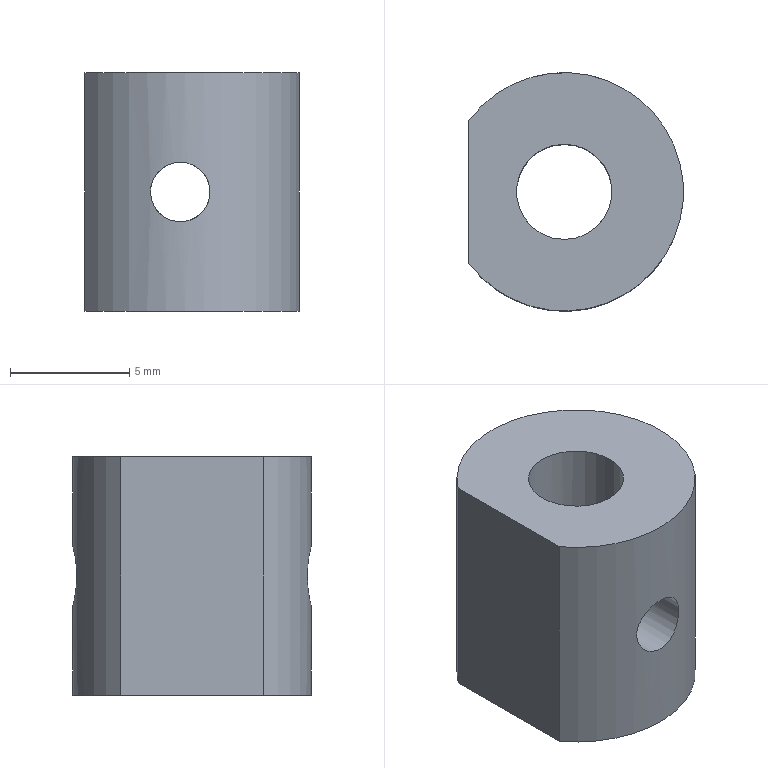Component | NX | 22B__27_2 | 1 solid | 7 faces | volume 589 mm3 | cylinder 4 | plane 3 | commonest cylinder face diameters 2.5 x2 10 x1 4 x1